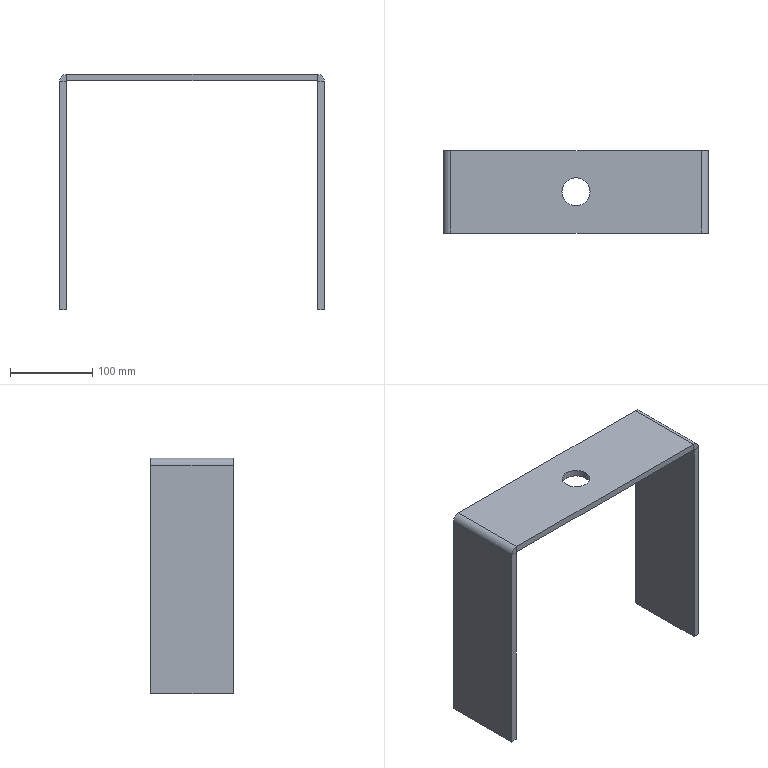Component | SolidWorks | CounterweightFixingFrame-1 | 1 solid | 24 faces | box 321 x 100 x 286 mm | volume 691084 mm3 | plane 18 | cylinder 6 | commonest cylinder face diameters 34 x2 17.473 x2 1.473 x2 | material Q235
STEP:
#1=COLOUR_RGB('',0.7922,0.8196,0.9333);
#2=FILL_AREA_STYLE_COLOUR('',#1);
#3=FILL_AREA_STYLE('',(#2));
#4=SURFACE_STYLE_FILL_AREA(#3);
#5=SURFACE_SIDE_STYLE('',(#4));
#6=SURFACE_STYLE_USAGE(.BOTH.,#5);
#7=PRESENTATION_STYLE_ASSIGNMENT((#6));
#8=CARTESIAN_POINT('',(-33.057,28.719,106.17));
#9=VERTEX_POINT('',#8);
#10=CARTESIAN_POINT('',(-31.719,28.719,106.17));
#11=VERTEX_POINT('',#10);
#12=CARTESIAN_POINT('',(-32.388,28.719,106.17));
#13=DIRECTION('',(0.,0.,-1.));
#14=DIRECTION('',(1.,0.,0.));
#15=AXIS2_PLACEMENT_3D('',#12,#13,#14);
#16=CIRCLE('',#15,0.6693);
#17=EDGE_CURVE('',#9,#11,#16,.T.);
#18=ORIENTED_EDGE('',*,*,#17,.T.);
#19=CARTESIAN_POINT('',(-31.719,28.719,106.485));
#20=VERTEX_POINT('',#19);
#21=CARTESIAN_POINT('',(-31.719,28.719,106.091));
#22=DIRECTION('',(-0.,-0.,1.));
#23=VECTOR('',#22,39.37);
#24=LINE('',#21,#23);
#25=EDGE_CURVE('',#11,#20,#24,.T.);
#26=ORIENTED_EDGE('',*,*,#25,.T.);
#27=CARTESIAN_POINT('',(-33.057,28.719,106.485));
#28=VERTEX_POINT('',#27);
#29=CARTESIAN_POINT('',(-32.388,28.719,106.485));
#30=DIRECTION('',(-0.,-0.,1.));
#31=DIRECTION('',(-1.,0.,0.));
#32=AXIS2_PLACEMENT_3D('',#29,#30,#31);
#33=CIRCLE('',#32,0.6693);
#34=EDGE_CURVE('',#20,#28,#33,.T.);
#35=ORIENTED_EDGE('',*,*,#34,.T.);
#36=CARTESIAN_POINT('',(-33.057,28.719,106.091));
#37=DIRECTION('',(-0.,-0.,1.));
#38=VECTOR('',#37,39.37);
#39=LINE('',#36,#38);
#40=EDGE_CURVE('',#9,#28,#39,.T.);
#41=ORIENTED_EDGE('',*,*,#40,.F.);
#42=EDGE_LOOP('',(#18,#26,#35,#41));
#43=FACE_OUTER_BOUND('',#42,.T.);
#44=CARTESIAN_POINT('',(-32.388,28.719,106.091));
#45=DIRECTION('',(-0.,-0.,1.));
#46=DIRECTION('',(-1.,0.,0.));
#47=AXIS2_PLACEMENT_3D('',#44,#45,#46);
#48=CYLINDRICAL_SURFACE('',#47,0.6693);
#49=ADVANCED_FACE('',(#43),#48,.F.);
#50=CARTESIAN_POINT('',(-32.388,28.719,106.485));
#51=DIRECTION('',(-0.,-0.,1.));
#52=DIRECTION('',(-1.,0.,0.));
#53=AXIS2_PLACEMENT_3D('',#50,#51,#52);
#54=CIRCLE('',#53,0.6693);
#55=EDGE_CURVE('',#28,#20,#54,.T.);
#56=ORIENTED_EDGE('',*,*,#55,.F.);
#57=ORIENTED_EDGE('',*,*,#34,.F.);
#58=EDGE_LOOP('',(#56,#57));
#59=FACE_BOUND('',#58,.T.);
#60=CARTESIAN_POINT('',(-26.413,26.751,106.485));
#61=VERTEX_POINT('',#60);
#62=CARTESIAN_POINT('',(-26.413,30.688,106.485));
#63=VERTEX_POINT('',#62);
#64=CARTESIAN_POINT('',(-26.413,26.751,106.485));
#65=DIRECTION('',(0.,1.,0.));
#66=VECTOR('',#65,39.37);
#67=LINE('',#64,#66);
#68=EDGE_CURVE('',#61,#63,#67,.T.);
#69=ORIENTED_EDGE('',*,*,#68,.T.);
#70=CARTESIAN_POINT('',(-38.363,30.688,106.485));
#71=VERTEX_POINT('',#70);
#72=CARTESIAN_POINT('',(-38.707,30.688,106.485));
#73=DIRECTION('',(1.,-0.,0.));
#74=VECTOR('',#73,39.37);
#75=LINE('',#72,#74);
#76=EDGE_CURVE('',#71,#63,#75,.T.);
#77=ORIENTED_EDGE('',*,*,#76,.F.);
#78=CARTESIAN_POINT('',(-38.363,26.751,106.485));
#79=VERTEX_POINT('',#78);
#80=CARTESIAN_POINT('',(-38.363,30.688,106.485));
#81=DIRECTION('',(-0.,-1.,-0.));
#82=VECTOR('',#81,39.37);
#83=LINE('',#80,#82);
#84=EDGE_CURVE('',#71,#79,#83,.T.);
#85=ORIENTED_EDGE('',*,*,#84,.T.);
#86=CARTESIAN_POINT('',(-38.707,26.751,106.485));
#87=DIRECTION('',(-1.,0.,-0.));
#88=VECTOR('',#87,39.37);
#89=LINE('',#86,#88);
#90=EDGE_CURVE('',#61,#79,#89,.T.);
#91=ORIENTED_EDGE('',*,*,#90,.F.);
#92=EDGE_LOOP('',(#69,#77,#85,#91));
#93=FACE_OUTER_BOUND('',#92,.T.);
#94=CARTESIAN_POINT('',(-32.388,28.719,106.485));
#95=DIRECTION('',(0.,0.,-1.));
#96=DIRECTION('',(1.,-0.,0.));
#97=AXIS2_PLACEMENT_3D('',#94,#95,#96);
#98=PLANE('',#97);
#99=ADVANCED_FACE('',(#59,#93),#98,.F.);
#100=ORIENTED_EDGE('',*,*,#17,.F.);
#101=CARTESIAN_POINT('',(-32.388,28.719,106.17));
#102=DIRECTION('',(0.,0.,-1.));
#103=DIRECTION('',(1.,0.,0.));
#104=AXIS2_PLACEMENT_3D('',#101,#102,#103);
#105=CIRCLE('',#104,0.6693);
#106=EDGE_CURVE('',#11,#9,#105,.T.);
#107=ORIENTED_EDGE('',*,*,#106,.F.);
#108=EDGE_LOOP('',(#100,#107));
#109=FACE_BOUND('',#108,.T.);
#110=CARTESIAN_POINT('',(-38.363,30.688,106.17));
#111=VERTEX_POINT('',#110);
#112=CARTESIAN_POINT('',(-26.413,30.688,106.17));
#113=VERTEX_POINT('',#112);
#114=CARTESIAN_POINT('',(-38.707,30.688,106.17));
#115=DIRECTION('',(1.,-0.,0.));
#116=VECTOR('',#115,39.37);
#117=LINE('',#114,#116);
#118=EDGE_CURVE('',#111,#113,#117,.T.);
#119=ORIENTED_EDGE('',*,*,#118,.T.);
#120=CARTESIAN_POINT('',(-26.413,26.751,106.17));
#121=VERTEX_POINT('',#120);
#122=CARTESIAN_POINT('',(-26.413,26.751,106.17));
#123=DIRECTION('',(0.,1.,0.));
#124=VECTOR('',#123,39.37);
#125=LINE('',#122,#124);
#126=EDGE_CURVE('',#121,#113,#125,.T.);
#127=ORIENTED_EDGE('',*,*,#126,.F.);
#128=CARTESIAN_POINT('',(-38.363,26.751,106.17));
#129=VERTEX_POINT('',#128);
#130=CARTESIAN_POINT('',(-38.707,26.751,106.17));
#131=DIRECTION('',(-1.,0.,-0.));
#132=VECTOR('',#131,39.37);
#133=LINE('',#130,#132);
#134=EDGE_CURVE('',#121,#129,#133,.T.);
#135=ORIENTED_EDGE('',*,*,#134,.T.);
#136=CARTESIAN_POINT('',(-38.363,30.688,106.17));
#137=DIRECTION('',(-0.,-1.,-0.));
#138=VECTOR('',#137,39.37);
#139=LINE('',#136,#138);
#140=EDGE_CURVE('',#111,#129,#139,.T.);
#141=ORIENTED_EDGE('',*,*,#140,.F.);
#142=EDGE_LOOP('',(#119,#127,#135,#141));
#143=FACE_OUTER_BOUND('',#142,.T.);
#144=CARTESIAN_POINT('',(-32.388,28.719,106.17));
#145=DIRECTION('',(0.,0.,-1.));
#146=DIRECTION('',(1.,-0.,0.));
#147=AXIS2_PLACEMENT_3D('',#144,#145,#146);
#148=PLANE('',#147);
#149=ADVANCED_FACE('',(#109,#143),#148,.T.);
#150=ORIENTED_EDGE('',*,*,#134,.F.);
#151=CARTESIAN_POINT('',(-26.413,26.751,106.17));
#152=DIRECTION('',(-0.,-0.,1.));
#153=VECTOR('',#152,39.37);
#154=LINE('',#151,#153);
#155=EDGE_CURVE('',#121,#61,#154,.T.);
#156=ORIENTED_EDGE('',*,*,#155,.T.);
#157=ORIENTED_EDGE('',*,*,#90,.T.);
#158=CARTESIAN_POINT('',(-38.363,26.751,106.17));
#159=DIRECTION('',(-0.,-0.,1.));
#160=VECTOR('',#159,39.37);
#161=LINE('',#158,#160);
#162=EDGE_CURVE('',#129,#79,#161,.T.);
#163=ORIENTED_EDGE('',*,*,#162,.F.);
#164=EDGE_LOOP('',(#150,#156,#157,#163));
#165=FACE_OUTER_BOUND('',#164,.T.);
#166=CARTESIAN_POINT('',(-38.707,26.751,106.485));
#167=DIRECTION('',(-0.,-1.,-0.));
#168=DIRECTION('',(0.,0.,-1.));
#169=AXIS2_PLACEMENT_3D('',#166,#167,#168);
#170=PLANE('',#169);
#171=ADVANCED_FACE('',(#165),#170,.T.);
#172=CARTESIAN_POINT('',(-26.413,30.688,106.17));
#173=DIRECTION('',(-0.,-0.,1.));
#174=VECTOR('',#173,39.37);
#175=LINE('',#172,#174);
#176=EDGE_CURVE('',#113,#63,#175,.T.);
#177=ORIENTED_EDGE('',*,*,#176,.F.);
#178=ORIENTED_EDGE('',*,*,#118,.F.);
#179=CARTESIAN_POINT('',(-38.363,30.688,106.17));
#180=DIRECTION('',(-0.,-0.,1.));
#181=VECTOR('',#180,39.37);
#182=LINE('',#179,#181);
#183=EDGE_CURVE('',#111,#71,#182,.T.);
#184=ORIENTED_EDGE('',*,*,#183,.T.);
#185=ORIENTED_EDGE('',*,*,#76,.T.);
#186=EDGE_LOOP('',(#177,#178,#184,#185));
#187=FACE_OUTER_BOUND('',#186,.T.);
#188=CARTESIAN_POINT('',(-38.707,30.688,106.485));
#189=DIRECTION('',(0.,1.,0.));
#190=DIRECTION('',(-0.,-0.,1.));
#191=AXIS2_PLACEMENT_3D('',#188,#189,#190);
#192=PLANE('',#191);
#193=ADVANCED_FACE('',(#187),#192,.T.);
#194=CARTESIAN_POINT('',(-38.392,26.751,106.141));
#195=VERTEX_POINT('',#194);
#196=CARTESIAN_POINT('',(-38.707,26.751,106.141));
#197=VERTEX_POINT('',#196);
#198=CARTESIAN_POINT('',(-38.707,26.751,106.141));
#199=DIRECTION('',(-1.,0.,-0.));
#200=VECTOR('',#199,39.37);
#201=LINE('',#198,#200);
#202=EDGE_CURVE('',#195,#197,#201,.T.);
#203=ORIENTED_EDGE('',*,*,#202,.F.);
#204=CARTESIAN_POINT('',(-38.363,26.751,106.141));
#205=DIRECTION('',(-0.,-1.,-0.));
#206=DIRECTION('',(0.,0.,1.));
#207=AXIS2_PLACEMENT_3D('',#204,#205,#206);
#208=CIRCLE('',#207,0.029);
#209=EDGE_CURVE('',#129,#195,#208,.T.);
#210=ORIENTED_EDGE('',*,*,#209,.F.);
#211=ORIENTED_EDGE('',*,*,#162,.T.);
#212=CARTESIAN_POINT('',(-38.363,26.751,106.141));
#213=DIRECTION('',(-0.,-1.,-0.));
#214=DIRECTION('',(0.,0.,1.));
#215=AXIS2_PLACEMENT_3D('',#212,#213,#214);
#216=CIRCLE('',#215,0.344);
#217=EDGE_CURVE('',#79,#197,#216,.T.);
#218=ORIENTED_EDGE('',*,*,#217,.T.);
#219=EDGE_LOOP('',(#203,#210,#211,#218));
#220=FACE_OUTER_BOUND('',#219,.T.);
#221=CARTESIAN_POINT('',(-38.363,26.751,106.141));
#222=DIRECTION('',(-0.,-1.,-0.));
#223=DIRECTION('',(0.,0.,-1.));
#224=AXIS2_PLACEMENT_3D('',#221,#222,#223);
#225=PLANE('',#224);
#226=ADVANCED_FACE('',(#220),#225,.T.);
#227=CARTESIAN_POINT('',(-38.392,30.688,106.141));
#228=VERTEX_POINT('',#227);
#229=CARTESIAN_POINT('',(-38.363,30.688,106.141));
#230=DIRECTION('',(0.,1.,0.));
#231=DIRECTION('',(0.,0.,1.));
#232=AXIS2_PLACEMENT_3D('',#229,#230,#231);
#233=CIRCLE('',#232,0.029);
#234=EDGE_CURVE('',#228,#111,#233,.T.);
#235=ORIENTED_EDGE('',*,*,#234,.F.);
#236=CARTESIAN_POINT('',(-38.707,30.688,106.141));
#237=VERTEX_POINT('',#236);
#238=CARTESIAN_POINT('',(-38.392,30.688,106.141));
#239=DIRECTION('',(-1.,0.,-0.));
#240=VECTOR('',#239,39.37);
#241=LINE('',#238,#240);
#242=EDGE_CURVE('',#228,#237,#241,.T.);
#243=ORIENTED_EDGE('',*,*,#242,.T.);
#244=CARTESIAN_POINT('',(-38.363,30.688,106.141));
#245=DIRECTION('',(0.,1.,0.));
#246=DIRECTION('',(-0.,0.,1.));
#247=AXIS2_PLACEMENT_3D('',#244,#245,#246);
#248=CIRCLE('',#247,0.344);
#249=EDGE_CURVE('',#237,#71,#248,.T.);
#250=ORIENTED_EDGE('',*,*,#249,.T.);
#251=ORIENTED_EDGE('',*,*,#183,.F.);
#252=EDGE_LOOP('',(#235,#243,#250,#251));
#253=FACE_OUTER_BOUND('',#252,.T.);
#254=CARTESIAN_POINT('',(-38.363,30.688,106.141));
#255=DIRECTION('',(-0.,-1.,-0.));
#256=DIRECTION('',(0.,0.,-1.));
#257=AXIS2_PLACEMENT_3D('',#254,#255,#256);
#258=PLANE('',#257);
#259=ADVANCED_FACE('',(#253),#258,.F.);
#260=ORIENTED_EDGE('',*,*,#84,.F.);
#261=ORIENTED_EDGE('',*,*,#249,.F.);
#262=CARTESIAN_POINT('',(-38.707,28.719,106.141));
#263=DIRECTION('',(0.,1.,0.));
#264=VECTOR('',#263,39.37);
#265=LINE('',#262,#264);
#266=EDGE_CURVE('',#197,#237,#265,.T.);
#267=ORIENTED_EDGE('',*,*,#266,.F.);
#268=ORIENTED_EDGE('',*,*,#217,.F.);
#269=EDGE_LOOP('',(#260,#261,#267,#268));
#270=FACE_OUTER_BOUND('',#269,.T.);
#271=CARTESIAN_POINT('',(-38.363,30.688,106.141));
#272=DIRECTION('',(0.,1.,0.));
#273=DIRECTION('',(-1.,0.,0.));
#274=AXIS2_PLACEMENT_3D('',#271,#272,#273);
#275=CYLINDRICAL_SURFACE('',#274,0.344);
#276=ADVANCED_FACE('',(#270),#275,.T.);
#277=ORIENTED_EDGE('',*,*,#140,.T.);
#278=ORIENTED_EDGE('',*,*,#209,.T.);
#279=CARTESIAN_POINT('',(-38.392,26.751,106.141));
#280=DIRECTION('',(0.,1.,0.));
#281=VECTOR('',#280,39.37);
#282=LINE('',#279,#281);
#283=EDGE_CURVE('',#195,#228,#282,.T.);
#284=ORIENTED_EDGE('',*,*,#283,.T.);
#285=ORIENTED_EDGE('',*,*,#234,.T.);
#286=EDGE_LOOP('',(#277,#278,#284,#285));
#287=FACE_OUTER_BOUND('',#286,.T.);
#288=CARTESIAN_POINT('',(-38.363,30.688,106.141));
#289=DIRECTION('',(0.,1.,0.));
#290=DIRECTION('',(-1.,0.,0.));
#291=AXIS2_PLACEMENT_3D('',#288,#289,#290);
#292=CYLINDRICAL_SURFACE('',#291,0.029);
#293=ADVANCED_FACE('',(#287),#292,.F.);
#294=CARTESIAN_POINT('',(-38.707,30.688,95.225));
#295=VERTEX_POINT('',#294);
#296=CARTESIAN_POINT('',(-38.707,30.688,106.17));
#297=DIRECTION('',(-0.,-0.,1.));
#298=VECTOR('',#297,39.37);
#299=LINE('',#296,#298);
#300=EDGE_CURVE('',#295,#237,#299,.T.);
#301=ORIENTED_EDGE('',*,*,#300,.T.);
#302=ORIENTED_EDGE('',*,*,#242,.F.);
#303=CARTESIAN_POINT('',(-38.392,30.688,95.225));
#304=VERTEX_POINT('',#303);
#305=CARTESIAN_POINT('',(-38.392,30.688,106.17));
#306=DIRECTION('',(-0.,-0.,1.));
#307=VECTOR('',#306,39.37);
#308=LINE('',#305,#307);
#309=EDGE_CURVE('',#304,#228,#308,.T.);
#310=ORIENTED_EDGE('',*,*,#309,.F.);
#311=CARTESIAN_POINT('',(-38.707,30.688,95.225));
#312=DIRECTION('',(1.,-0.,0.));
#313=VECTOR('',#312,39.37);
#314=LINE('',#311,#313);
#315=EDGE_CURVE('',#295,#304,#314,.T.);
#316=ORIENTED_EDGE('',*,*,#315,.F.);
#317=EDGE_LOOP('',(#301,#302,#310,#316));
#318=FACE_OUTER_BOUND('',#317,.T.);
#319=CARTESIAN_POINT('',(-38.707,30.688,106.17));
#320=DIRECTION('',(0.,1.,0.));
#321=DIRECTION('',(-0.,-0.,1.));
#322=AXIS2_PLACEMENT_3D('',#319,#320,#321);
#323=PLANE('',#322);
#324=ADVANCED_FACE('',(#318),#323,.T.);
#325=CARTESIAN_POINT('',(-38.392,26.751,95.225));
#326=VERTEX_POINT('',#325);
#327=CARTESIAN_POINT('',(-38.392,26.751,106.17));
#328=DIRECTION('',(0.,0.,-1.));
#329=VECTOR('',#328,39.37);
#330=LINE('',#327,#329);
#331=EDGE_CURVE('',#195,#326,#330,.T.);
#332=ORIENTED_EDGE('',*,*,#331,.F.);
#333=ORIENTED_EDGE('',*,*,#202,.T.);
#334=CARTESIAN_POINT('',(-38.707,26.751,95.225));
#335=VERTEX_POINT('',#334);
#336=CARTESIAN_POINT('',(-38.707,26.751,95.225));
#337=DIRECTION('',(0.,0.,-1.));
#338=VECTOR('',#337,39.37);
#339=LINE('',#336,#338);
#340=EDGE_CURVE('',#197,#335,#339,.T.);
#341=ORIENTED_EDGE('',*,*,#340,.T.);
#342=CARTESIAN_POINT('',(-38.707,26.751,95.225));
#343=DIRECTION('',(1.,-0.,0.));
#344=VECTOR('',#343,39.37);
#345=LINE('',#342,#344);
#346=EDGE_CURVE('',#335,#326,#345,.T.);
#347=ORIENTED_EDGE('',*,*,#346,.T.);
#348=EDGE_LOOP('',(#332,#333,#341,#347));
#349=FACE_OUTER_BOUND('',#348,.T.);
#350=CARTESIAN_POINT('',(-38.707,26.751,95.225));
#351=DIRECTION('',(-0.,-1.,-0.));
#352=DIRECTION('',(0.,0.,-1.));
#353=AXIS2_PLACEMENT_3D('',#350,#351,#352);
#354=PLANE('',#353);
#355=ADVANCED_FACE('',(#349),#354,.T.);
#356=ORIENTED_EDGE('',*,*,#340,.F.);
#357=ORIENTED_EDGE('',*,*,#266,.T.);
#358=ORIENTED_EDGE('',*,*,#300,.F.);
#359=CARTESIAN_POINT('',(-38.707,30.688,95.225));
#360=DIRECTION('',(0.,1.,0.));
#361=VECTOR('',#360,39.37);
#362=LINE('',#359,#361);
#363=EDGE_CURVE('',#335,#295,#362,.T.);
#364=ORIENTED_EDGE('',*,*,#363,.F.);
#365=EDGE_LOOP('',(#356,#357,#358,#364));
#366=FACE_OUTER_BOUND('',#365,.T.);
#367=CARTESIAN_POINT('',(-38.707,28.719,106.17));
#368=DIRECTION('',(-1.,0.,-0.));
#369=DIRECTION('',(0.,0.,-1.));
#370=AXIS2_PLACEMENT_3D('',#367,#368,#369);
#371=PLANE('',#370);
#372=ADVANCED_FACE('',(#366),#371,.T.);
#373=ORIENTED_EDGE('',*,*,#283,.F.);
#374=ORIENTED_EDGE('',*,*,#331,.T.);
#375=CARTESIAN_POINT('',(-38.392,28.719,95.225));
#376=DIRECTION('',(0.,1.,0.));
#377=VECTOR('',#376,39.37);
#378=LINE('',#375,#377);
#379=EDGE_CURVE('',#326,#304,#378,.T.);
#380=ORIENTED_EDGE('',*,*,#379,.T.);
#381=ORIENTED_EDGE('',*,*,#309,.T.);
#382=EDGE_LOOP('',(#373,#374,#380,#381));
#383=FACE_OUTER_BOUND('',#382,.T.);
#384=CARTESIAN_POINT('',(-38.392,28.719,106.17));
#385=DIRECTION('',(-1.,0.,-0.));
#386=DIRECTION('',(0.,0.,-1.));
#387=AXIS2_PLACEMENT_3D('',#384,#385,#386);
#388=PLANE('',#387);
#389=ADVANCED_FACE('',(#383),#388,.F.);
#390=ORIENTED_EDGE('',*,*,#379,.F.);
#391=ORIENTED_EDGE('',*,*,#346,.F.);
#392=ORIENTED_EDGE('',*,*,#363,.T.);
#393=ORIENTED_EDGE('',*,*,#315,.T.);
#394=EDGE_LOOP('',(#390,#391,#392,#393));
#395=FACE_OUTER_BOUND('',#394,.T.);
#396=CARTESIAN_POINT('',(-38.707,30.688,95.225));
#397=DIRECTION('',(0.,0.,-1.));
#398=DIRECTION('',(1.,-0.,0.));
#399=AXIS2_PLACEMENT_3D('',#396,#397,#398);
#400=PLANE('',#399);
#401=ADVANCED_FACE('',(#395),#400,.T.);
#402=CARTESIAN_POINT('',(-26.384,30.688,106.141));
#403=VERTEX_POINT('',#402);
#404=CARTESIAN_POINT('',(-26.069,30.688,106.141));
#405=VERTEX_POINT('',#404);
#406=CARTESIAN_POINT('',(-26.069,30.688,106.141));
#407=DIRECTION('',(1.,-0.,0.));
#408=VECTOR('',#407,39.37);
#409=LINE('',#406,#408);
#410=EDGE_CURVE('',#403,#405,#409,.T.);
#411=ORIENTED_EDGE('',*,*,#410,.F.);
#412=CARTESIAN_POINT('',(-26.413,30.688,106.141));
#413=DIRECTION('',(0.,1.,0.));
#414=DIRECTION('',(0.,0.,-1.));
#415=AXIS2_PLACEMENT_3D('',#412,#413,#414);
#416=CIRCLE('',#415,0.029);
#417=EDGE_CURVE('',#113,#403,#416,.T.);
#418=ORIENTED_EDGE('',*,*,#417,.F.);
#419=ORIENTED_EDGE('',*,*,#176,.T.);
#420=CARTESIAN_POINT('',(-26.413,30.688,106.141));
#421=DIRECTION('',(0.,1.,0.));
#422=DIRECTION('',(0.,0.,-1.));
#423=AXIS2_PLACEMENT_3D('',#420,#421,#422);
#424=CIRCLE('',#423,0.344);
#425=EDGE_CURVE('',#63,#405,#424,.T.);
#426=ORIENTED_EDGE('',*,*,#425,.T.);
#427=EDGE_LOOP('',(#411,#418,#419,#426));
#428=FACE_OUTER_BOUND('',#427,.T.);
#429=CARTESIAN_POINT('',(-26.413,30.688,106.141));
#430=DIRECTION('',(0.,1.,0.));
#431=DIRECTION('',(-0.,-0.,1.));
#432=AXIS2_PLACEMENT_3D('',#429,#430,#431);
#433=PLANE('',#432);
#434=ADVANCED_FACE('',(#428),#433,.T.);
#435=CARTESIAN_POINT('',(-26.384,26.751,106.141));
#436=VERTEX_POINT('',#435);
#437=CARTESIAN_POINT('',(-26.413,26.751,106.141));
#438=DIRECTION('',(-0.,-1.,-0.));
#439=DIRECTION('',(0.,0.,-1.));
#440=AXIS2_PLACEMENT_3D('',#437,#438,#439);
#441=CIRCLE('',#440,0.029);
#442=EDGE_CURVE('',#436,#121,#441,.T.);
#443=ORIENTED_EDGE('',*,*,#442,.F.);
#444=CARTESIAN_POINT('',(-26.069,26.751,106.141));
#445=VERTEX_POINT('',#444);
#446=CARTESIAN_POINT('',(-26.384,26.751,106.141));
#447=DIRECTION('',(1.,-0.,0.));
#448=VECTOR('',#447,39.37);
#449=LINE('',#446,#448);
#450=EDGE_CURVE('',#436,#445,#449,.T.);
#451=ORIENTED_EDGE('',*,*,#450,.T.);
#452=CARTESIAN_POINT('',(-26.413,26.751,106.141));
#453=DIRECTION('',(-0.,-1.,-0.));
#454=DIRECTION('',(0.,0.,-1.));
#455=AXIS2_PLACEMENT_3D('',#452,#453,#454);
#456=CIRCLE('',#455,0.344);
#457=EDGE_CURVE('',#445,#61,#456,.T.);
#458=ORIENTED_EDGE('',*,*,#457,.T.);
#459=ORIENTED_EDGE('',*,*,#155,.F.);
#460=EDGE_LOOP('',(#443,#451,#458,#459));
#461=FACE_OUTER_BOUND('',#460,.T.);
#462=CARTESIAN_POINT('',(-26.413,26.751,106.141));
#463=DIRECTION('',(0.,1.,0.));
#464=DIRECTION('',(-0.,-0.,1.));
#465=AXIS2_PLACEMENT_3D('',#462,#463,#464);
#466=PLANE('',#465);
#467=ADVANCED_FACE('',(#461),#466,.F.);
#468=ORIENTED_EDGE('',*,*,#68,.F.);
#469=ORIENTED_EDGE('',*,*,#457,.F.);
#470=CARTESIAN_POINT('',(-26.069,28.719,106.141));
#471=DIRECTION('',(-0.,-1.,-0.));
#472=VECTOR('',#471,39.37);
#473=LINE('',#470,#472);
#474=EDGE_CURVE('',#405,#445,#473,.T.);
#475=ORIENTED_EDGE('',*,*,#474,.F.);
#476=ORIENTED_EDGE('',*,*,#425,.F.);
#477=EDGE_LOOP('',(#468,#469,#475,#476));
#478=FACE_OUTER_BOUND('',#477,.T.);
#479=CARTESIAN_POINT('',(-26.413,26.751,106.141));
#480=DIRECTION('',(-0.,-1.,-0.));
#481=DIRECTION('',(1.,0.,0.));
#482=AXIS2_PLACEMENT_3D('',#479,#480,#481);
#483=CYLINDRICAL_SURFACE('',#482,0.344);
#484=ADVANCED_FACE('',(#478),#483,.T.);
#485=ORIENTED_EDGE('',*,*,#126,.T.);
#486=ORIENTED_EDGE('',*,*,#417,.T.);
#487=CARTESIAN_POINT('',(-26.384,30.688,106.141));
#488=DIRECTION('',(-0.,-1.,-0.));
#489=VECTOR('',#488,39.37);
#490=LINE('',#487,#489);
#491=EDGE_CURVE('',#403,#436,#490,.T.);
#492=ORIENTED_EDGE('',*,*,#491,.T.);
#493=ORIENTED_EDGE('',*,*,#442,.T.);
#494=EDGE_LOOP('',(#485,#486,#492,#493));
#495=FACE_OUTER_BOUND('',#494,.T.);
#496=CARTESIAN_POINT('',(-26.413,26.751,106.141));
#497=DIRECTION('',(-0.,-1.,-0.));
#498=DIRECTION('',(1.,0.,0.));
#499=AXIS2_PLACEMENT_3D('',#496,#497,#498);
#500=CYLINDRICAL_SURFACE('',#499,0.029);
#501=ADVANCED_FACE('',(#495),#500,.F.);
#502=CARTESIAN_POINT('',(-26.069,26.751,95.225));
#503=VERTEX_POINT('',#502);
#504=CARTESIAN_POINT('',(-26.069,26.751,106.17));
#505=DIRECTION('',(-0.,-0.,1.));
#506=VECTOR('',#505,39.37);
#507=LINE('',#504,#506);
#508=EDGE_CURVE('',#503,#445,#507,.T.);
#509=ORIENTED_EDGE('',*,*,#508,.T.);
#510=ORIENTED_EDGE('',*,*,#450,.F.);
#511=CARTESIAN_POINT('',(-26.384,26.751,95.225));
#512=VERTEX_POINT('',#511);
#513=CARTESIAN_POINT('',(-26.384,26.751,106.17));
#514=DIRECTION('',(-0.,-0.,1.));
#515=VECTOR('',#514,39.37);
#516=LINE('',#513,#515);
#517=EDGE_CURVE('',#512,#436,#516,.T.);
#518=ORIENTED_EDGE('',*,*,#517,.F.);
#519=CARTESIAN_POINT('',(-26.069,26.751,95.225));
#520=DIRECTION('',(-1.,0.,-0.));
#521=VECTOR('',#520,39.37);
#522=LINE('',#519,#521);
#523=EDGE_CURVE('',#503,#512,#522,.T.);
#524=ORIENTED_EDGE('',*,*,#523,.F.);
#525=EDGE_LOOP('',(#509,#510,#518,#524));
#526=FACE_OUTER_BOUND('',#525,.T.);
#527=CARTESIAN_POINT('',(-26.069,26.751,106.17));
#528=DIRECTION('',(-0.,-1.,-0.));
#529=DIRECTION('',(0.,0.,-1.));
#530=AXIS2_PLACEMENT_3D('',#527,#528,#529);
#531=PLANE('',#530);
#532=ADVANCED_FACE('',(#526),#531,.T.);
#533=CARTESIAN_POINT('',(-26.384,30.688,95.225));
#534=VERTEX_POINT('',#533);
#535=CARTESIAN_POINT('',(-26.384,30.688,106.17));
#536=DIRECTION('',(0.,0.,-1.));
#537=VECTOR('',#536,39.37);
#538=LINE('',#535,#537);
#539=EDGE_CURVE('',#403,#534,#538,.T.);
#540=ORIENTED_EDGE('',*,*,#539,.F.);
#541=ORIENTED_EDGE('',*,*,#410,.T.);
#542=CARTESIAN_POINT('',(-26.069,30.688,95.225));
#543=VERTEX_POINT('',#542);
#544=CARTESIAN_POINT('',(-26.069,30.688,95.225));
#545=DIRECTION('',(0.,0.,-1.));
#546=VECTOR('',#545,39.37);
#547=LINE('',#544,#546);
#548=EDGE_CURVE('',#405,#543,#547,.T.);
#549=ORIENTED_EDGE('',*,*,#548,.T.);
#550=CARTESIAN_POINT('',(-26.069,30.688,95.225));
#551=DIRECTION('',(-1.,0.,-0.));
#552=VECTOR('',#551,39.37);
#553=LINE('',#550,#552);
#554=EDGE_CURVE('',#543,#534,#553,.T.);
#555=ORIENTED_EDGE('',*,*,#554,.T.);
#556=EDGE_LOOP('',(#540,#541,#549,#555));
#557=FACE_OUTER_BOUND('',#556,.T.);
#558=CARTESIAN_POINT('',(-26.069,30.688,95.225));
#559=DIRECTION('',(0.,1.,0.));
#560=DIRECTION('',(-0.,-0.,1.));
#561=AXIS2_PLACEMENT_3D('',#558,#559,#560);
#562=PLANE('',#561);
#563=ADVANCED_FACE('',(#557),#562,.T.);
#564=ORIENTED_EDGE('',*,*,#548,.F.);
#565=ORIENTED_EDGE('',*,*,#474,.T.);
#566=ORIENTED_EDGE('',*,*,#508,.F.);
#567=CARTESIAN_POINT('',(-26.069,26.751,95.225));
#568=DIRECTION('',(-0.,-1.,-0.));
#569=VECTOR('',#568,39.37);
#570=LINE('',#567,#569);
#571=EDGE_CURVE('',#543,#503,#570,.T.);
#572=ORIENTED_EDGE('',*,*,#571,.F.);
#573=EDGE_LOOP('',(#564,#565,#566,#572));
#574=FACE_OUTER_BOUND('',#573,.T.);
#575=CARTESIAN_POINT('',(-26.069,28.719,106.17));
#576=DIRECTION('',(1.,-0.,0.));
#577=DIRECTION('',(-0.,-0.,1.));
#578=AXIS2_PLACEMENT_3D('',#575,#576,#577);
#579=PLANE('',#578);
#580=ADVANCED_FACE('',(#574),#579,.T.);
#581=ORIENTED_EDGE('',*,*,#491,.F.);
#582=ORIENTED_EDGE('',*,*,#539,.T.);
#583=CARTESIAN_POINT('',(-26.384,28.719,95.225));
#584=DIRECTION('',(-0.,-1.,-0.));
#585=VECTOR('',#584,39.37);
#586=LINE('',#583,#585);
#587=EDGE_CURVE('',#534,#512,#586,.T.);
#588=ORIENTED_EDGE('',*,*,#587,.T.);
#589=ORIENTED_EDGE('',*,*,#517,.T.);
#590=EDGE_LOOP('',(#581,#582,#588,#589));
#591=FACE_OUTER_BOUND('',#590,.T.);
#592=CARTESIAN_POINT('',(-26.384,28.719,106.17));
#593=DIRECTION('',(1.,-0.,0.));
#594=DIRECTION('',(-0.,-0.,1.));
#595=AXIS2_PLACEMENT_3D('',#592,#593,#594);
#596=PLANE('',#595);
#597=ADVANCED_FACE('',(#591),#596,.F.);
#598=ORIENTED_EDGE('',*,*,#587,.F.);
#599=ORIENTED_EDGE('',*,*,#554,.F.);
#600=ORIENTED_EDGE('',*,*,#571,.T.);
#601=ORIENTED_EDGE('',*,*,#523,.T.);
#602=EDGE_LOOP('',(#598,#599,#600,#601));
#603=FACE_OUTER_BOUND('',#602,.T.);
#604=CARTESIAN_POINT('',(-26.069,26.751,95.225));
#605=DIRECTION('',(0.,0.,-1.));
#606=DIRECTION('',(1.,-0.,0.));
#607=AXIS2_PLACEMENT_3D('',#604,#605,#606);
#608=PLANE('',#607);
#609=ADVANCED_FACE('',(#603),#608,.T.);
#610=ORIENTED_EDGE('',*,*,#25,.F.);
#611=ORIENTED_EDGE('',*,*,#106,.T.);
#612=ORIENTED_EDGE('',*,*,#40,.T.);
#613=ORIENTED_EDGE('',*,*,#55,.T.);
#614=EDGE_LOOP('',(#610,#611,#612,#613));
#615=FACE_OUTER_BOUND('',#614,.T.);
#616=CARTESIAN_POINT('',(-32.388,28.719,106.091));
#617=DIRECTION('',(-0.,-0.,1.));
#618=DIRECTION('',(-1.,0.,0.));
#619=AXIS2_PLACEMENT_3D('',#616,#617,#618);
#620=CYLINDRICAL_SURFACE('',#619,0.6693);
#621=ADVANCED_FACE('',(#615),#620,.F.);
#622=CLOSED_SHELL('',(#49,#99,#149,#171,#193,#226,#259,#276,#293,#324,#355,#372,#389,#401,#434,#467,#484,#501,#532,#563,#580,#597,#609,#621));
#623=MANIFOLD_SOLID_BREP('',#622);
#624=STYLED_ITEM('',(#7),#623);
#625=(LENGTH_UNIT()NAMED_UNIT(*)SI_UNIT($,.METRE.));
#626=LENGTH_MEASURE_WITH_UNIT(LENGTH_MEASURE(0.0254),#625);
#627=DIMENSIONAL_EXPONENTS(1.,0.,0.,0.,0.,0.,0.);
#628=(CONVERSION_BASED_UNIT('',#626)LENGTH_UNIT()NAMED_UNIT(#627));
#629=UNCERTAINTY_MEASURE_WITH_UNIT(LENGTH_MEASURE(0.00001),#628,'','');
#630=(NAMED_UNIT(*)PLANE_ANGLE_UNIT()SI_UNIT($,.RADIAN.));
#631=(NAMED_UNIT(*)SI_UNIT($,.STERADIAN.)SOLID_ANGLE_UNIT());
#632=(GEOMETRIC_REPRESENTATION_CONTEXT(3)GLOBAL_UNCERTAINTY_ASSIGNED_CONTEXT((#629))GLOBAL_UNIT_ASSIGNED_CONTEXT((#628,#630,#631))REPRESENTATION_CONTEXT('',''));
#633=MECHANICAL_DESIGN_GEOMETRIC_PRESENTATION_REPRESENTATION('',(#624),#632);
#634=CARTESIAN_POINT('',(0.,0.,0.));
#635=DIRECTION('',(0.,0.,1.));
#636=DIRECTION('',(1.,0.,0.));
#637=AXIS2_PLACEMENT_3D('',#634,#635,#636);
#638=(LENGTH_UNIT()NAMED_UNIT(*)SI_UNIT($,.METRE.));
#639=LENGTH_MEASURE_WITH_UNIT(LENGTH_MEASURE(0.0254),#638);
#640=DIMENSIONAL_EXPONENTS(1.,0.,0.,0.,0.,0.,0.);
#641=(CONVERSION_BASED_UNIT('',#639)LENGTH_UNIT()NAMED_UNIT(#640));
#642=UNCERTAINTY_MEASURE_WITH_UNIT(LENGTH_MEASURE(0.00001),#641,'','');
#643=(NAMED_UNIT(*)PLANE_ANGLE_UNIT()SI_UNIT($,.RADIAN.));
#644=(NAMED_UNIT(*)SI_UNIT($,.STERADIAN.)SOLID_ANGLE_UNIT());
#645=(GEOMETRIC_REPRESENTATION_CONTEXT(3)GLOBAL_UNCERTAINTY_ASSIGNED_CONTEXT((#642))GLOBAL_UNIT_ASSIGNED_CONTEXT((#641,#643,#644))REPRESENTATION_CONTEXT('',''));
#646=ADVANCED_BREP_SHAPE_REPRESENTATION('',(#623,#637),#645);
#647=PRESENTATION_LAYER_ASSIGNMENT('','',(#624));